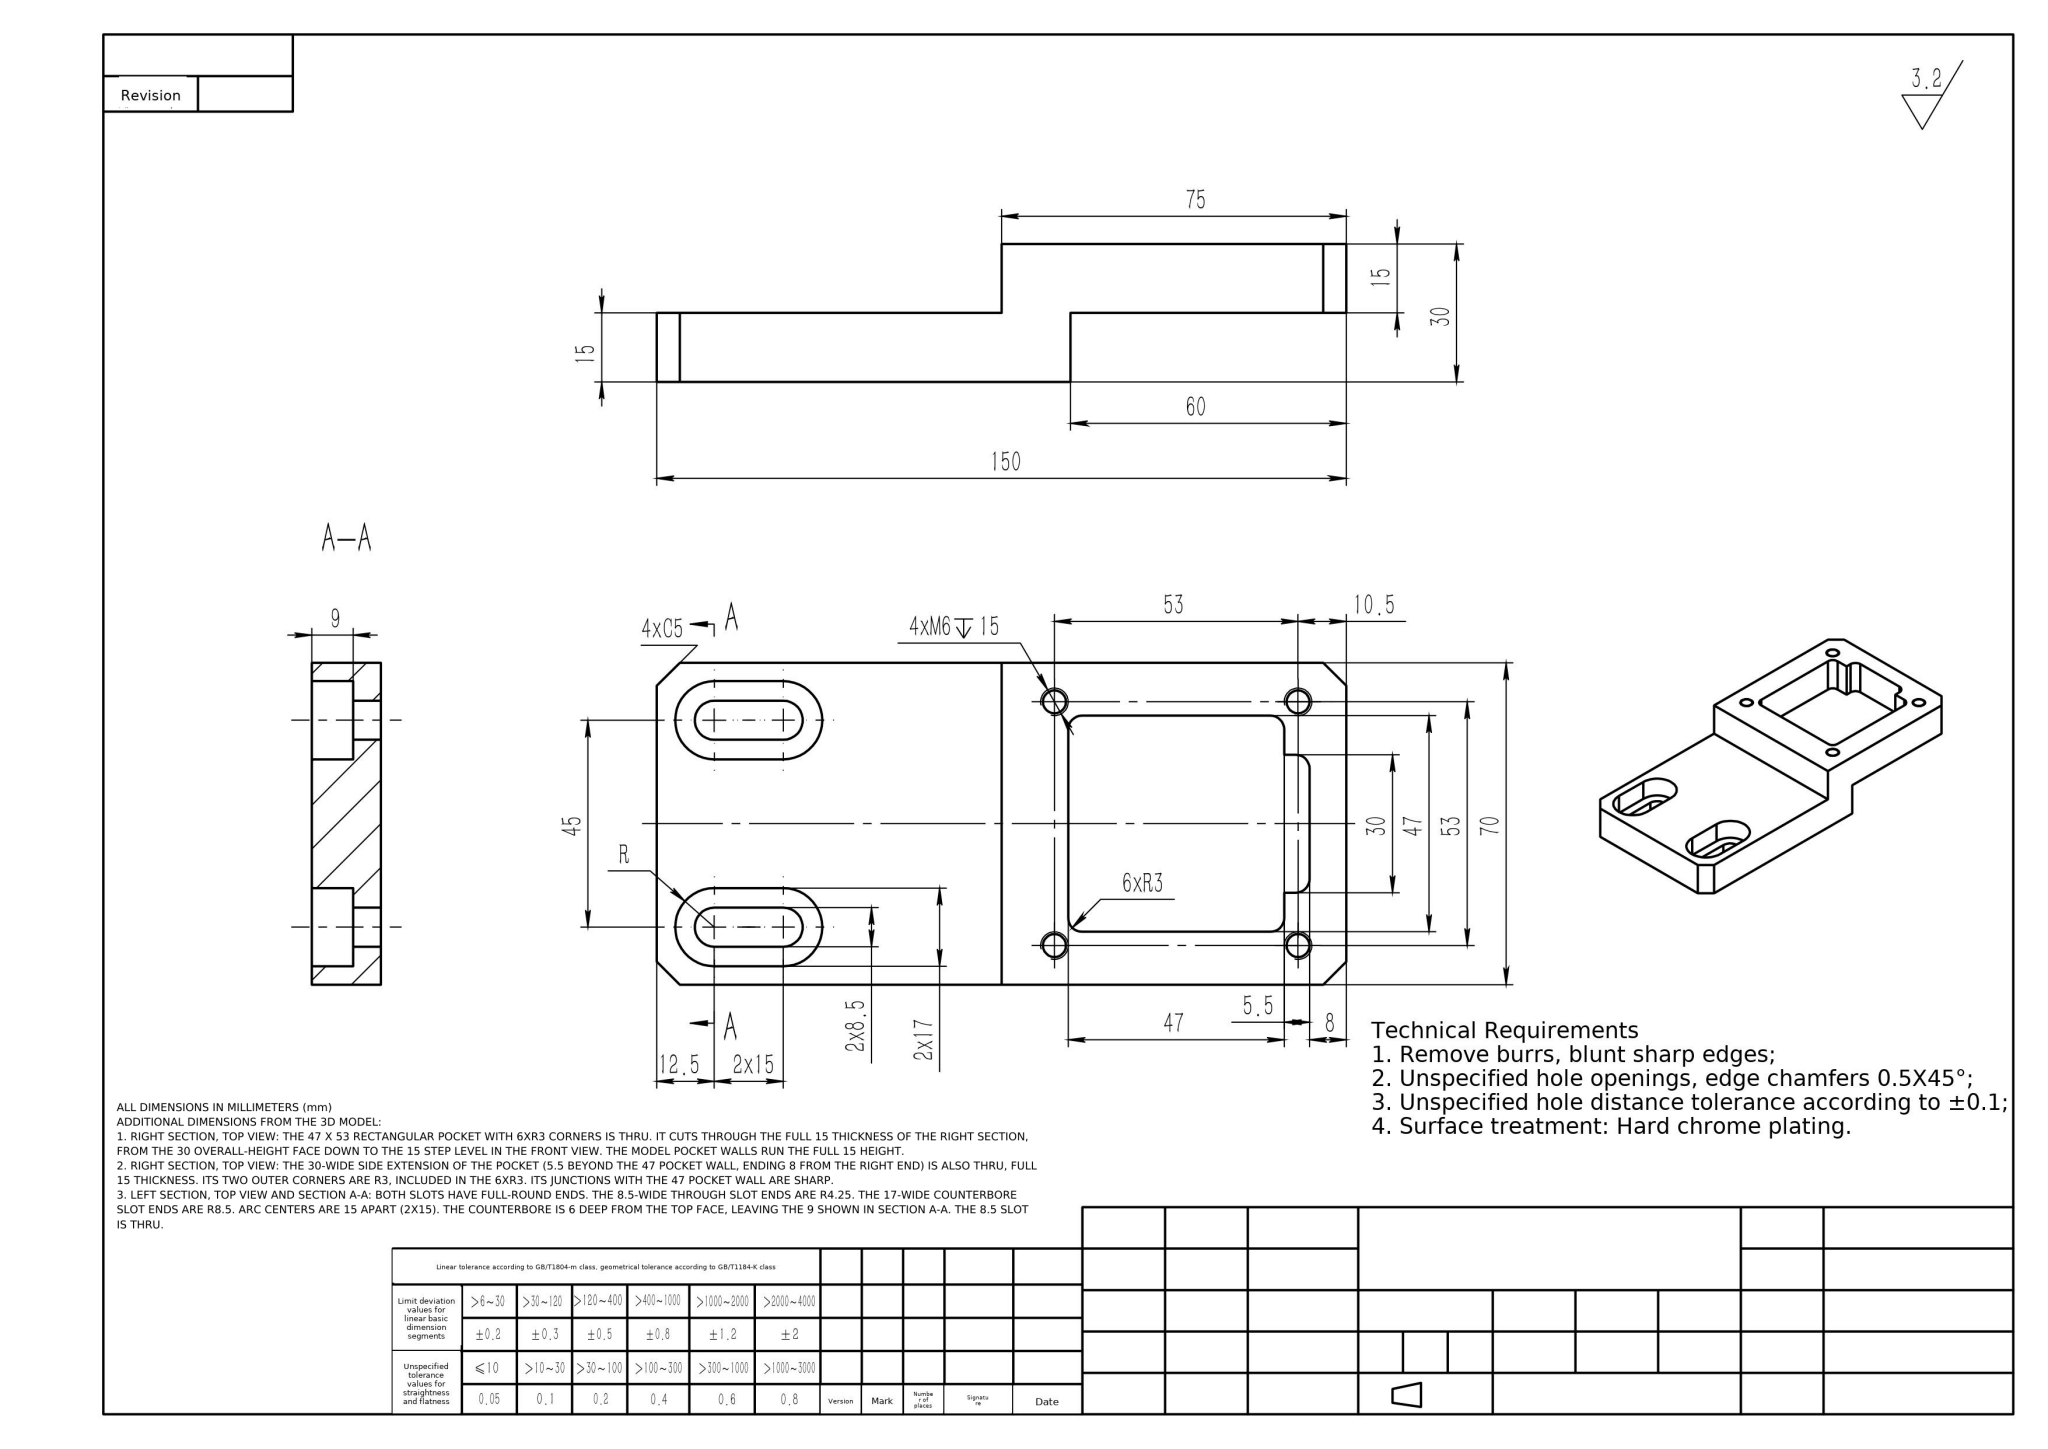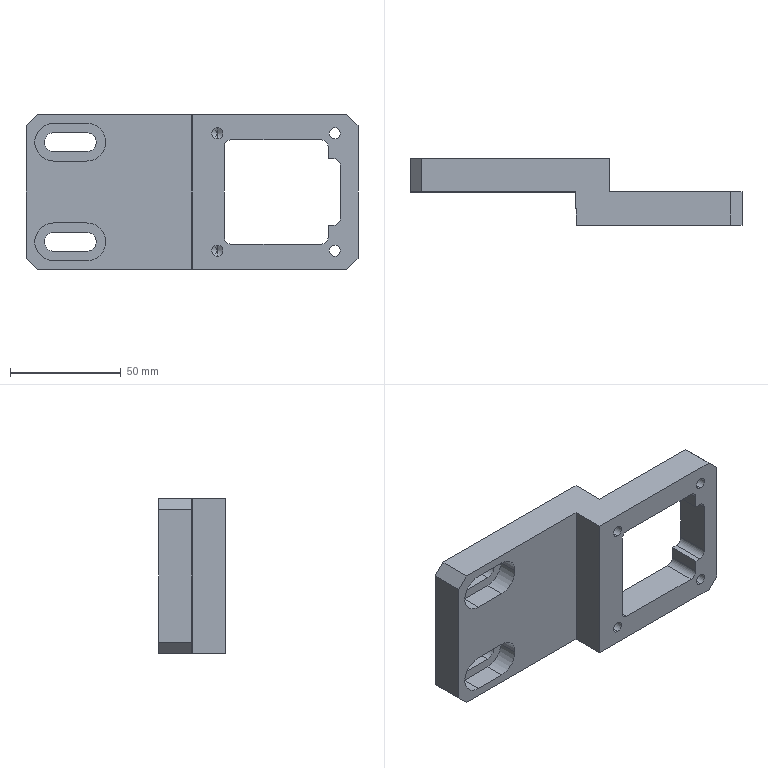Part | NX | mm | Notched Multi-Slot Corner Bracket | 1 solid | 63 faces | box 150 x 30 x 70 mm | volume 124655 mm3 | plane 33 | cylinder 26 | cone 4 | commonest cylinder face diameters 5 x8 17 x6 8.5 x6 6 x6